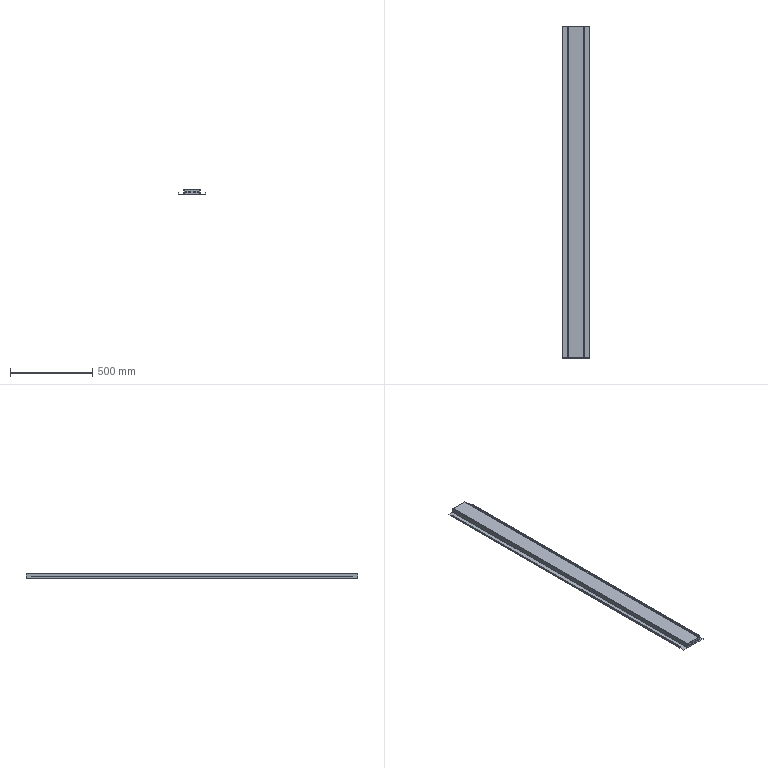Component | SolidWorks | MiddleColumn-1 | 1 solid | 98 faces | volume 728980 mm3 | plane 66 | cylinder 32 | commonest cylinder face diameters 11 x16 3.4 x8 0.4 x8